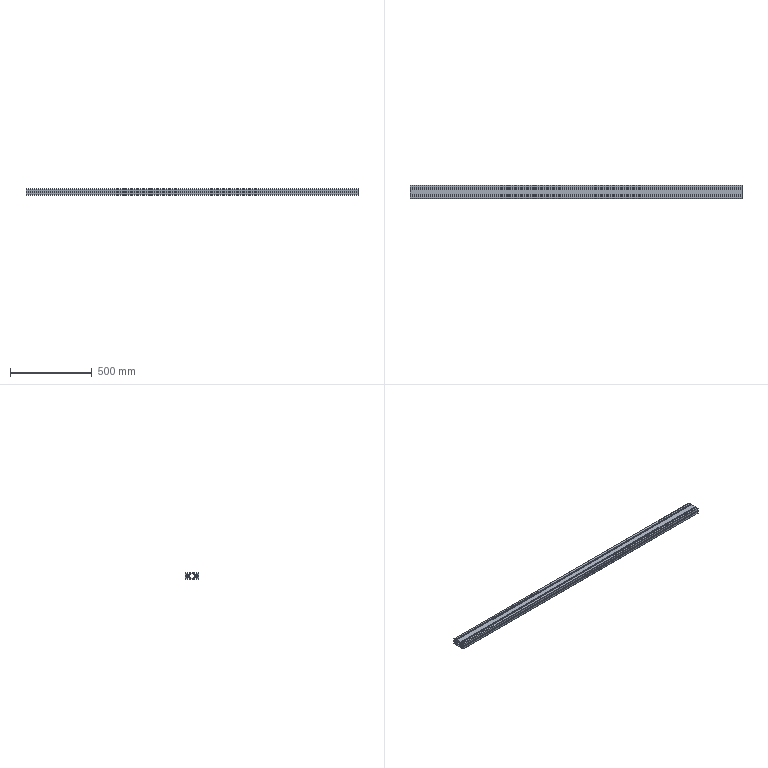Component | SolidWorks | Q1-GNFS8-4080-2030-2 | 1 solid | 130 faces | box 2030 x 80 x 40 mm | volume 2715830 mm3 | plane 106 | cylinder 24 | commonest cylinder face diameters 1 x13 6 x4 4 x4 10.5 x3 | material 6061
build123d program:
from build123d import *

# Parameters (mm, degrees)
MISUMI_ALUMINUM_EXTRUSION_GNFS8_4080_1_DEPTH = 2030


with BuildPart() as part:
    # Sketch11 → Misumi-Aluminum Extrusion GNFS8-4080_1 (new body)
    with BuildSketch(Plane.YZ):
        with BuildLine():
            Line((-17, -40), (-5, -40))
            Line((-5, -40), (-5, -34.5))
            Line((-5, -34.5), (-10, -34.5))
            Line((-10, -34.5), (-10, -31.768))
            Line((-10, -31.768), (-5.732, -27.5))
            Line((-5.732, -27.5), (-0.6536, -27.5))
            ThreePointArc((-0.6536, -27.5), (-0.5242, -27.483), (-0.4036, -27.433))
            Line((-0.4036, -27.433), (0, -27.2))
            Line((0, -27.2), (0.4036, -27.433))
            ThreePointArc((0.4036, -27.433), (0.6536, -27.5), (0.9036, -27.433))
            Line((0.9036, -27.433), (1.219, -27.251))
            Line((1.219, -27.251), (2.5, -27.5))
            Line((2.5, -27.5), (5.732, -27.5))
            Line((5.732, -27.5), (10, -31.768))
            Line((10, -31.768), (10, -34.5))
            Line((10, -34.5), (5, -34.5))
            Line((5, -34.5), (5, -40))
            Line((5, -40), (17, -40))
            ThreePointArc((17, -40), (19.121, -39.121), (20, -37))
            Line((20, -37), (20, -25))
            Line((20, -25), (14.5, -25))
            Line((14.5, -25), (14.5, -30))
            Line((14.5, -30), (11.768, -30))
            Line((11.768, -30), (7.5, -25.732))
            Line((7.5, -25.732), (7.5, -20.654))
            ThreePointArc((7.5, -20.654), (7.483, -20.524), (7.433, -20.404))
            Line((7.433, -20.404), (7.2, -20))
            Line((7.2, -20), (7.433, -19.596))
            ThreePointArc((7.433, -19.596), (7.5, -19.346), (7.433, -19.096))
            Line((7.433, -19.096), (7.251, -18.781))
            Line((7.251, -18.781), (7.5, -17.5))
            Line((7.5, -17.5), (7.5, -14.268))
            Line((7.5, -14.268), (11.768, -10))
            Line((11.768, -10), (14.5, -10))
            Line((14.5, -10), (14.5, -15))
            Line((14.5, -15), (20, -15))
            Line((20, -15), (20, 15))
            Line((20, 15), (14.5, 15))
            Line((14.5, 15), (14.5, 10))
            Line((14.5, 10), (11.768, 10))
            Line((11.768, 10), (7.5, 14.268))
            Line((7.5, 14.268), (7.5, 19.346))
            ThreePointArc((7.5, 19.346), (7.483, 19.476), (7.433, 19.596))
            Line((7.433, 19.596), (7.2, 20))
            Line((7.2, 20), (7.433, 20.404))
            ThreePointArc((7.433, 20.404), (7.5, 20.654), (7.433, 20.904))
            Line((7.433, 20.904), (7.251, 21.219))
            Line((7.251, 21.219), (7.5, 22.5))
            Line((7.5, 22.5), (7.5, 25.732))
            Line((7.5, 25.732), (11.768, 30))
            Line((11.768, 30), (14.5, 30))
            Line((14.5, 30), (14.5, 25))
            Line((14.5, 25), (20, 25))
            Line((20, 25), (20, 37))
            ThreePointArc((20, 37), (19.121, 39.121), (17, 40))
            Line((17, 40), (5, 40))
            Line((5, 40), (5, 34.5))
            Line((5, 34.5), (10, 34.5))
            Line((10, 34.5), (10, 31.768))
            Line((10, 31.768), (5.732, 27.5))
            Line((5.732, 27.5), (0.6536, 27.5))
            ThreePointArc((0.6536, 27.5), (0.5242, 27.483), (0.4036, 27.433))
            Line((0.4036, 27.433), (0, 27.2))
            Line((0, 27.2), (-0.4036, 27.433))
            ThreePointArc((-0.4036, 27.433), (-0.6536, 27.5), (-0.9036, 27.433))
            Line((-0.9036, 27.433), (-1.219, 27.251))
            Line((-1.219, 27.251), (-2.5, 27.5))
            Line((-2.5, 27.5), (-5.732, 27.5))
            Line((-5.732, 27.5), (-10, 31.768))
            Line((-10, 31.768), (-10, 34.5))
            Line((-10, 34.5), (-5, 34.5))
            Line((-5, 34.5), (-5, 40))
            Line((-5, 40), (-17, 40))
            ThreePointArc((-17, 40), (-19.121, 39.121), (-20, 37))
            Line((-20, 37), (-20, 25))
            Line((-20, 25), (-14.5, 25))
            Line((-14.5, 25), (-14.5, 30))
            Line((-14.5, 30), (-11.768, 30))
            Line((-11.768, 30), (-7.5, 25.732))
            Line((-7.5, 25.732), (-7.5, 20.654))
            ThreePointArc((-7.5, 20.654), (-7.483, 20.524), (-7.433, 20.404))
            Line((-7.433, 20.404), (-7.2, 20))
            Line((-7.2, 20), (-7.433, 19.596))
            ThreePointArc((-7.433, 19.596), (-7.5, 19.346), (-7.433, 19.096))
            Line((-7.433, 19.096), (-7.251, 18.781))
            Line((-7.251, 18.781), (-7.5, 17.5))
            Line((-7.5, 17.5), (-7.5, 14.268))
            Line((-7.5, 14.268), (-11.768, 10))
            Line((-11.768, 10), (-14.5, 10))
            Line((-14.5, 10), (-14.5, 15))
            Line((-14.5, 15), (-20, 15))
            Line((-20, 15), (-20, -15))
            Line((-20, -15), (-14.5, -15))
            Line((-14.5, -15), (-14.5, -10))
            Line((-14.5, -10), (-11.768, -10))
            Line((-11.768, -10), (-7.5, -14.268))
            Line((-7.5, -14.268), (-7.5, -19.346))
            ThreePointArc((-7.5, -19.346), (-7.483, -19.476), (-7.433, -19.596))
            Line((-7.433, -19.596), (-7.2, -20))
            Line((-7.2, -20), (-7.433, -20.404))
            ThreePointArc((-7.433, -20.404), (-7.5, -20.654), (-7.433, -20.904))
            Line((-7.433, -20.904), (-7.251, -21.219))
            Line((-7.251, -21.219), (-7.5, -22.5))
            Line((-7.5, -22.5), (-7.5, -25.732))
            Line((-7.5, -25.732), (-11.768, -30))
            Line((-11.768, -30), (-14.5, -30))
            Line((-14.5, -30), (-14.5, -25))
            Line((-14.5, -25), (-20, -25))
            Line((-20, -25), (-20, -37))
            ThreePointArc((-20, -37), (-19.121, -39.121), (-17, -40))
        make_face()
        with BuildLine():
            Line((-14.5, 7), (-14.5, -7))
            Line((-14.5, -7), (-10.525, -7))
            Line((-10.525, -7), (-3.886, -13.639))
            ThreePointArc((-3.886, -13.639), (-3.301, -15.019), (-3.838, -16.418))
            ThreePointArc((-3.838, -16.418), (0, -25.25), (3.838, -16.418))
            ThreePointArc((3.838, -16.418), (3.301, -15.019), (3.886, -13.639))
            Line((3.886, -13.639), (10.525, -7))
            Line((10.525, -7), (14.5, -7))
            Line((14.5, -7), (14.5, 7))
            Line((14.5, 7), (10.525, 7))
            Line((10.525, 7), (3.886, 13.639))
            ThreePointArc((3.886, 13.639), (3.301, 15.019), (3.838, 16.418))
            ThreePointArc((3.838, 16.418), (0, 25.25), (-3.838, 16.418))
            ThreePointArc((-3.838, 16.418), (-3.301, 15.019), (-3.886, 13.639))
            Line((-3.886, 13.639), (-10.525, 7))
            Line((-10.525, 7), (-14.5, 7))
        make_face(mode=Mode.SUBTRACT)
    extrude(amount=MISUMI_ALUMINUM_EXTRUSION_GNFS8_4080_1_DEPTH)


solid = part.part

# Placed as in the assembly
solid = solid.moved(Location((48.5, 0, -130), (90, 0, 0)))